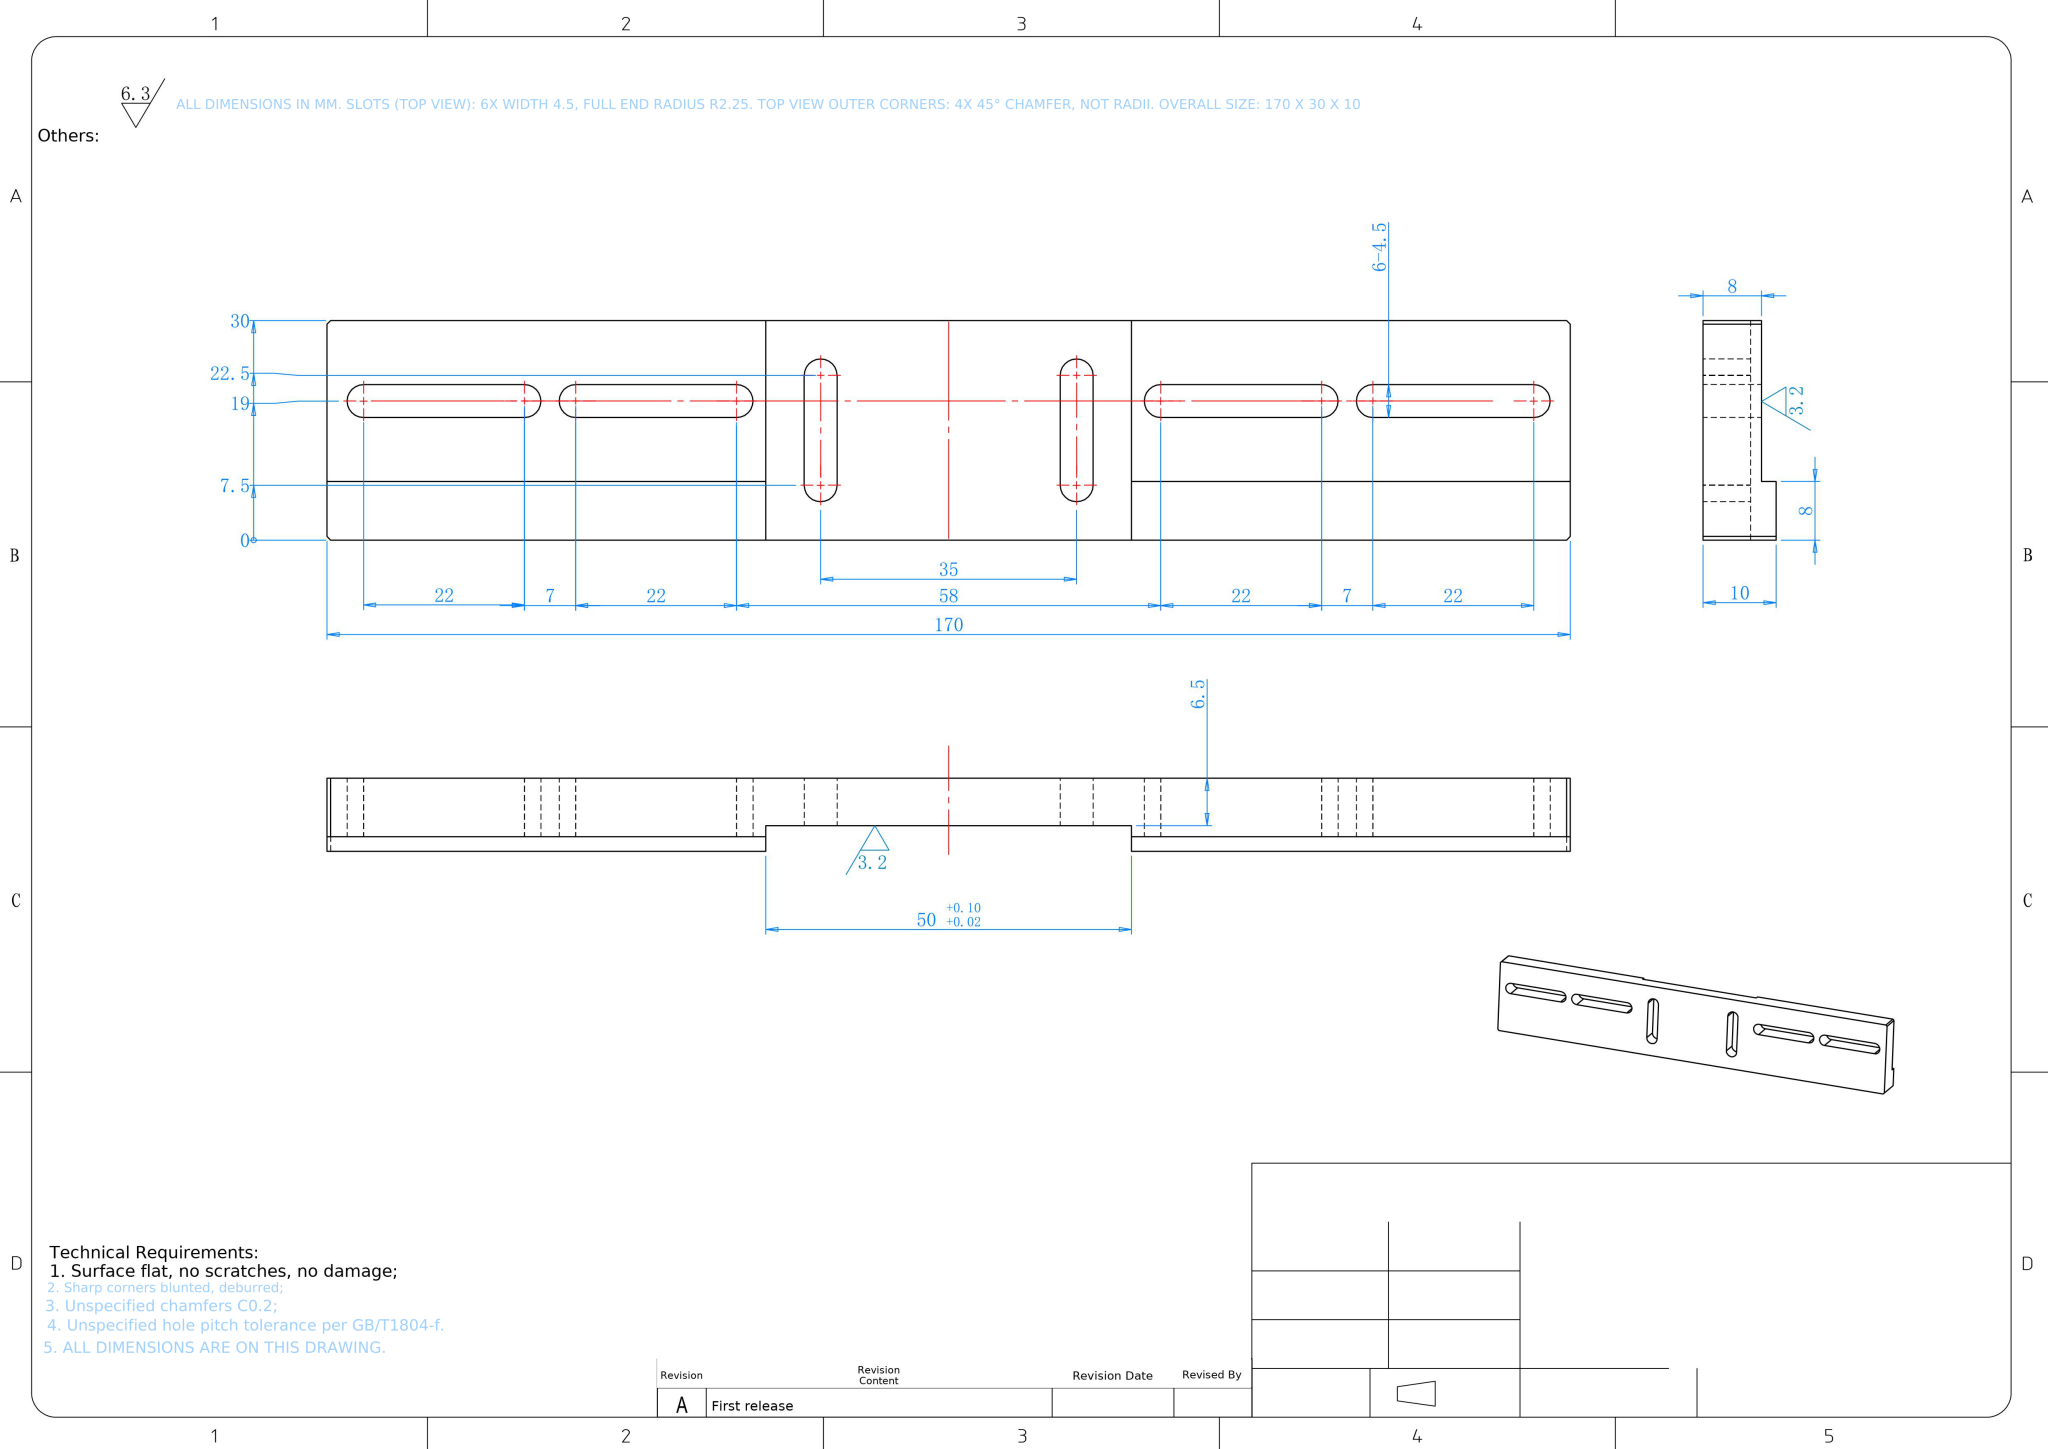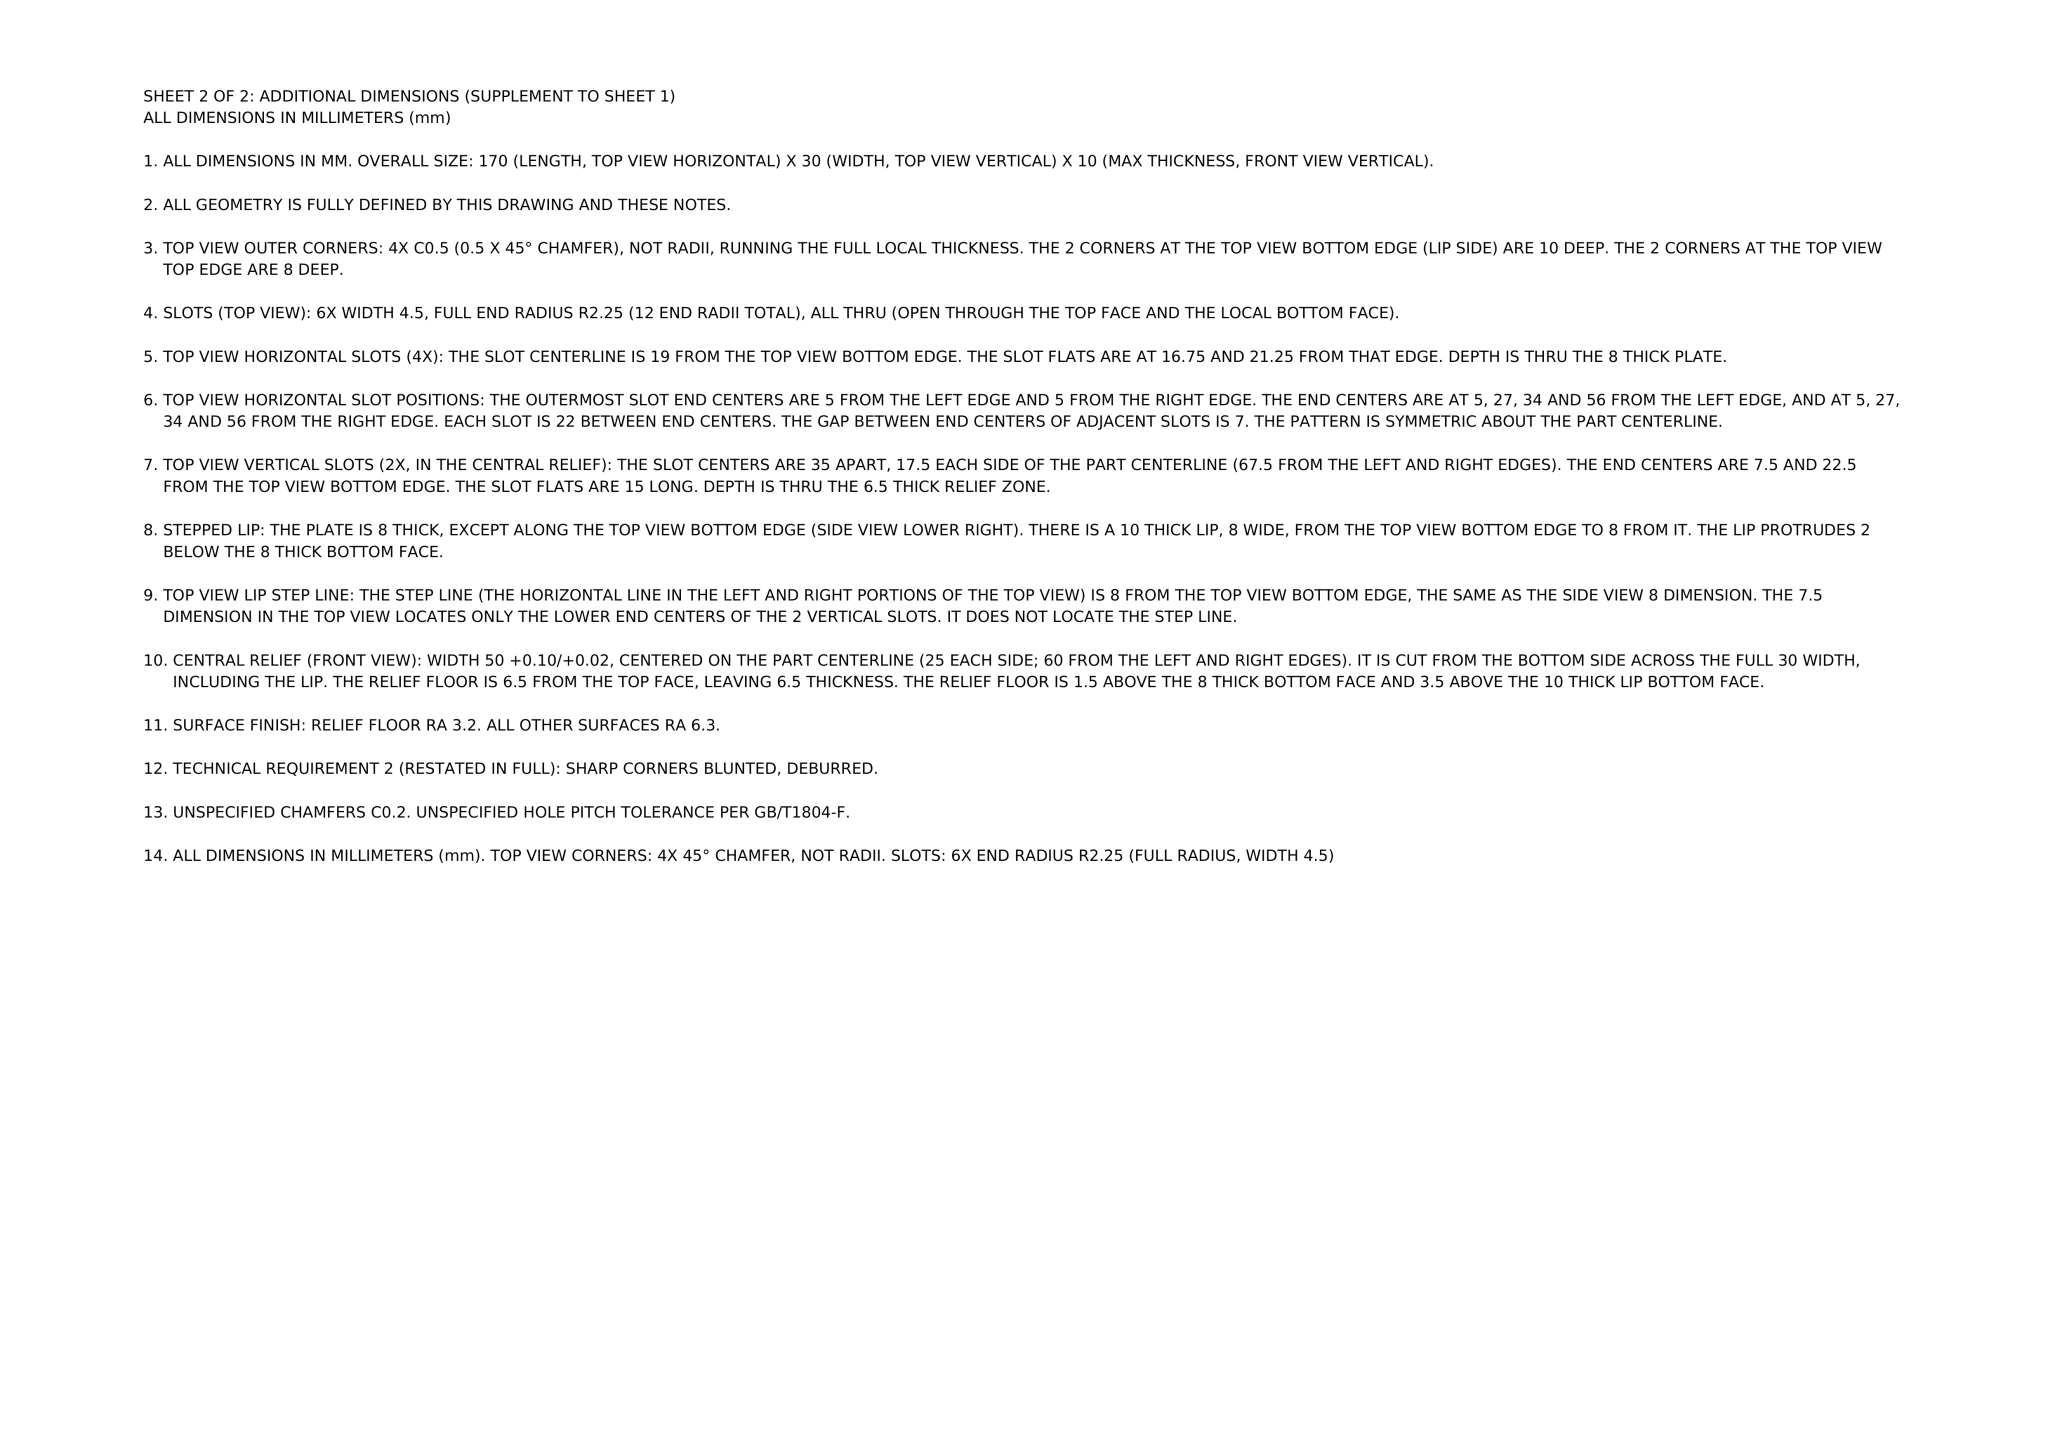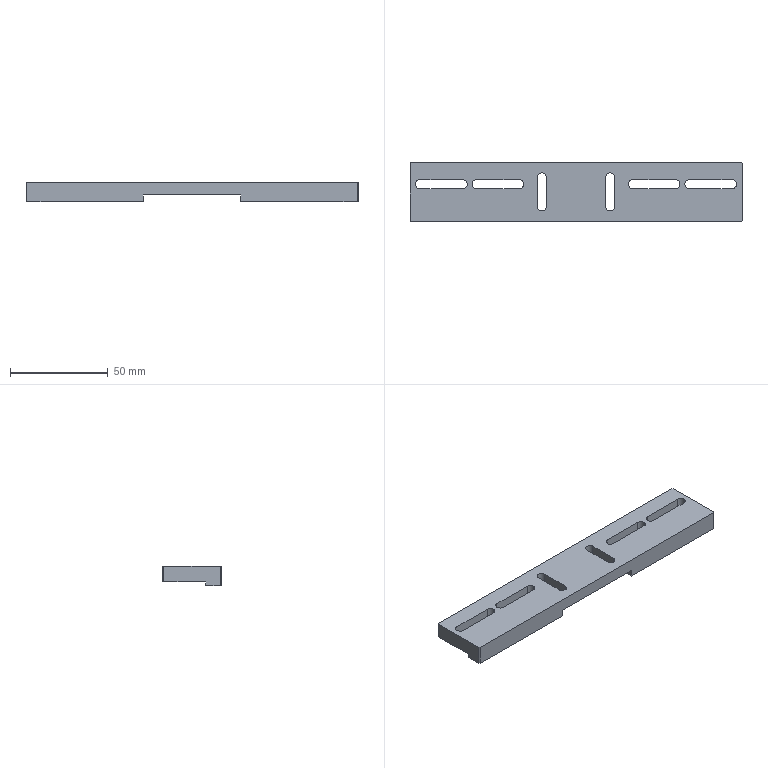Part | NX | mm | 1 solid | 46 faces | box 170 x 30 x 10 mm | volume 35704 mm3 | plane 30 | cylinder 16 | commonest cylinder face diameters 4.5 x16